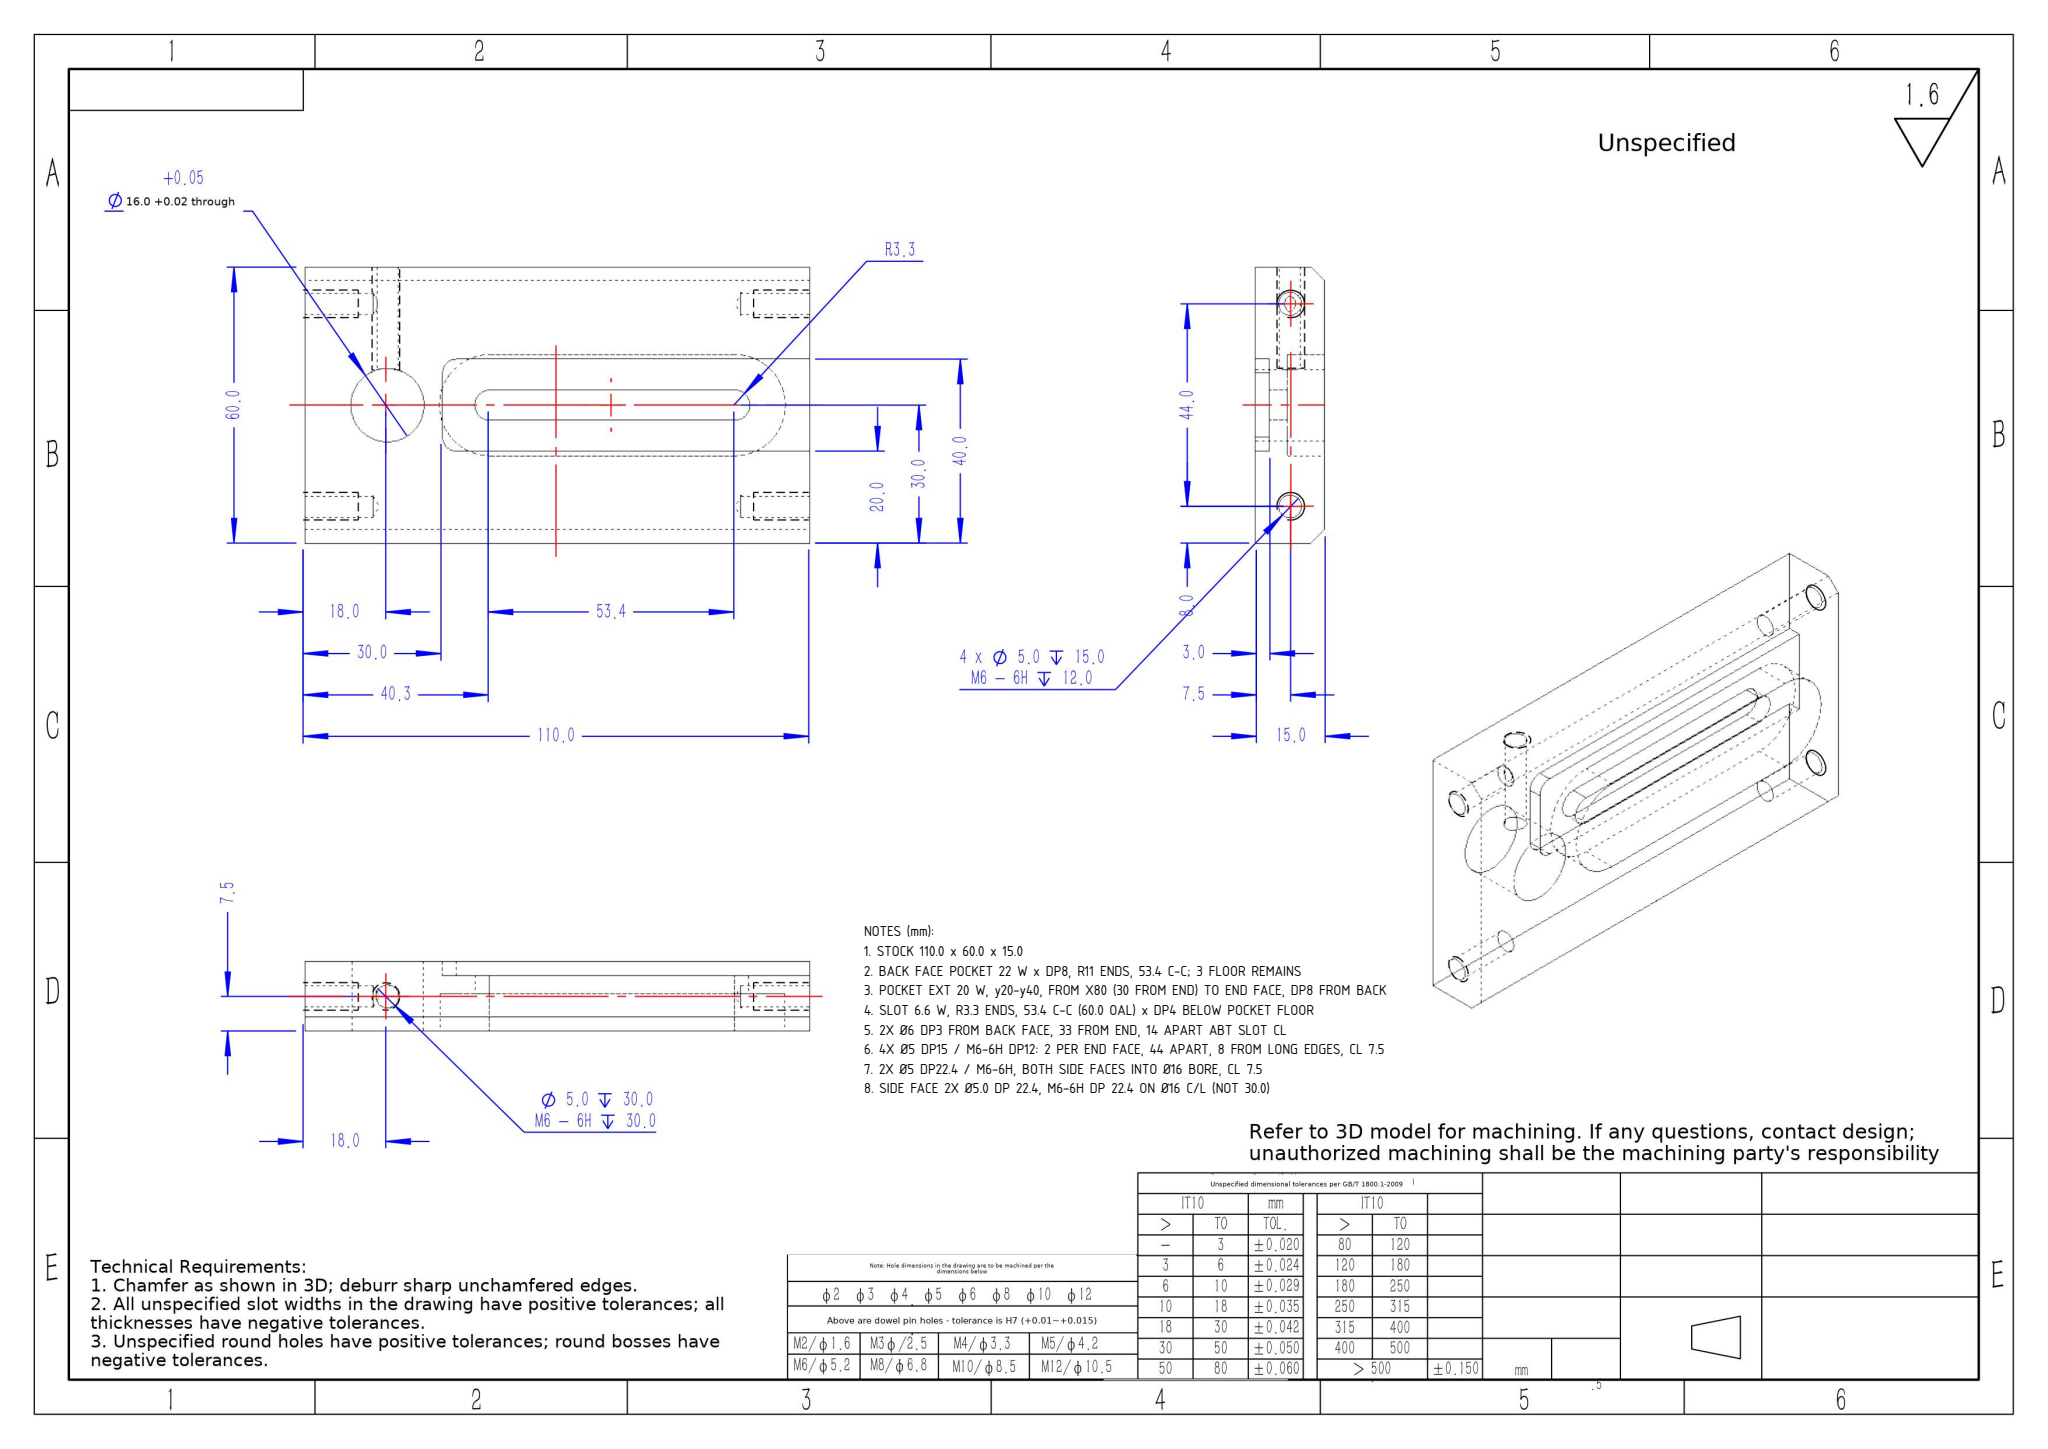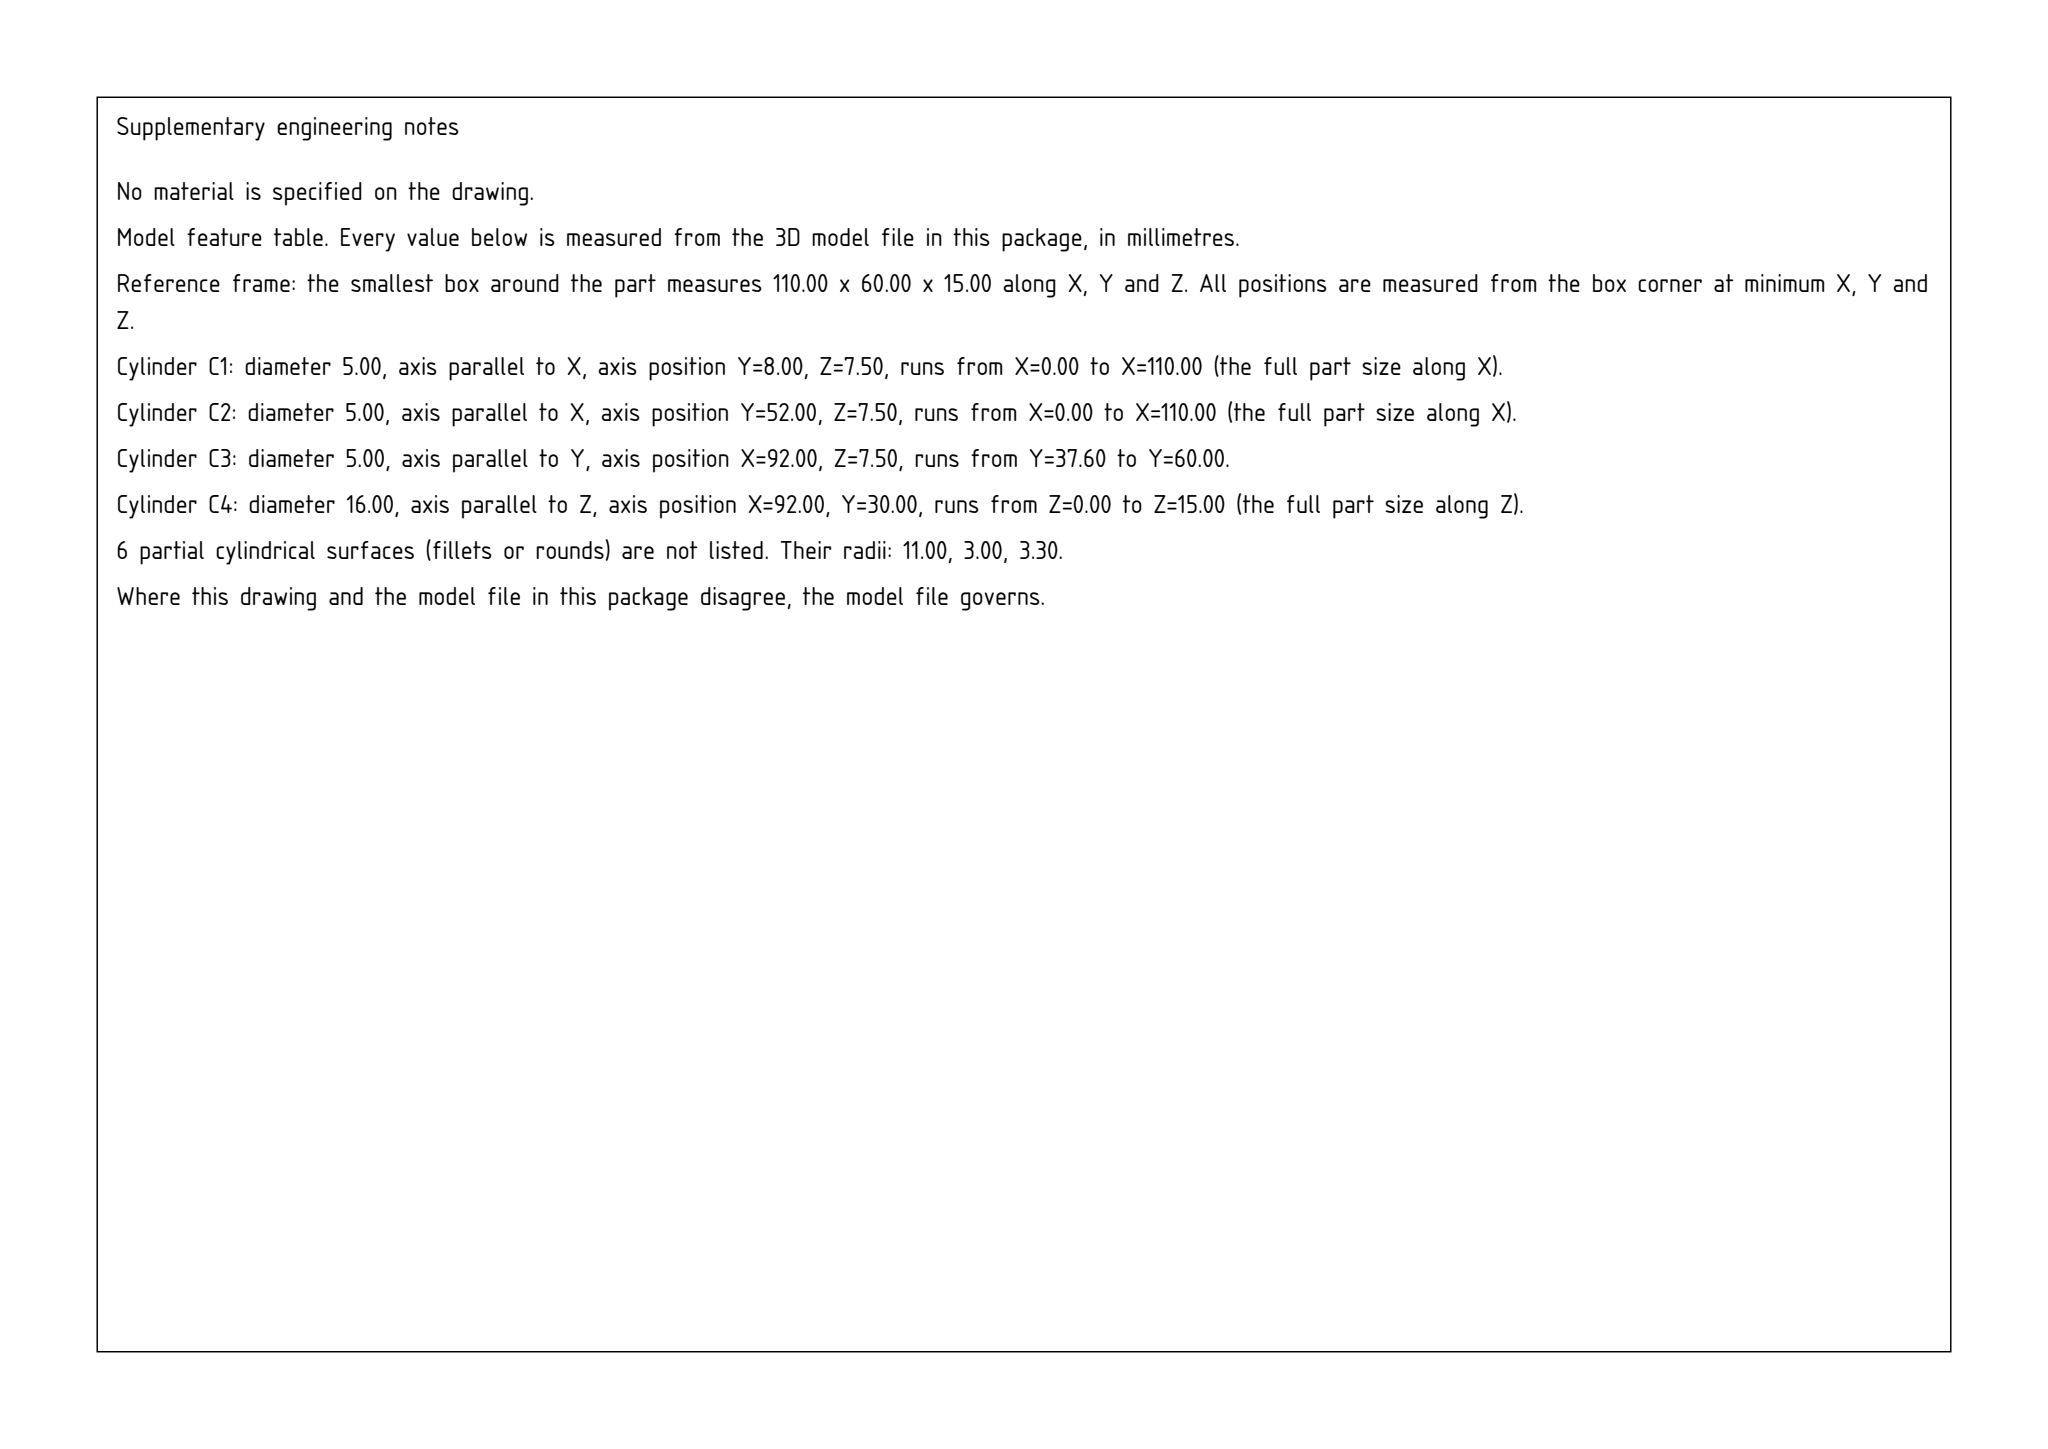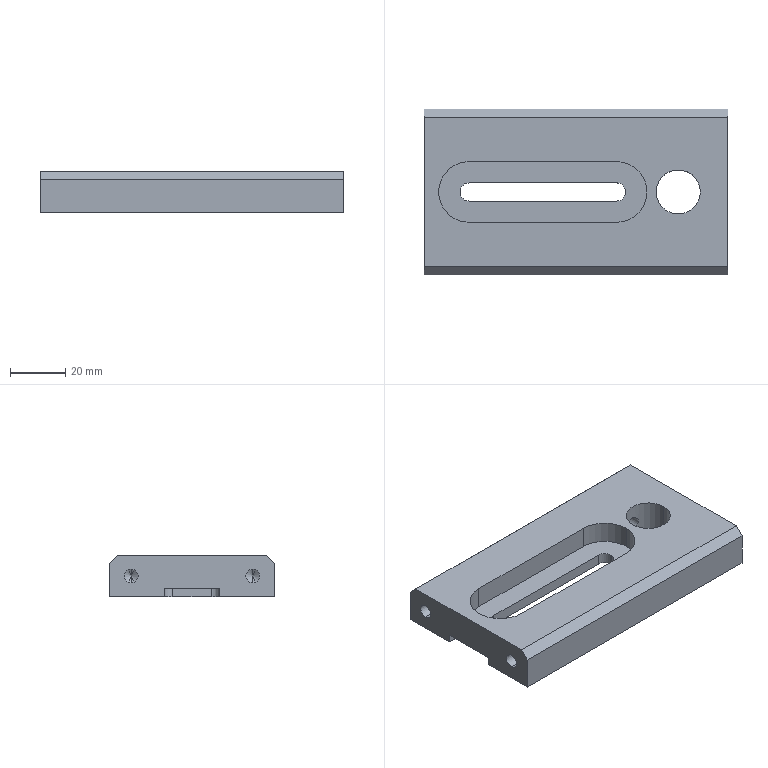Part | SolidWorks | mm | 1 solid | 45 faces | box 110 x 60 x 15 mm | volume 74570 mm3 | cylinder 20 | plane 17 | cone 8 | commonest cylinder face diameters 5 x10 22 x3 6.6 x3 16 x2 6 x2
Drawing notes:
STOCK 110.0 x 60.0 x 15.0 | from the solid: bbox_xyz [110,60,15]
BACK FACE POCKET 22 W x DP8, R11 ENDS, 53.4 C-C; 3 FLOOR REMAINS | from the solid: Ø22 z-cyls x=16.3 & 69.7 dp8; y-planes 19/41; z-planes 15 to 7; floor z0-3
POCKET EXT 20 W, y20-y40, FROM X80 (30 FROM END) TO END FACE, DP8 FROM BACK | from the solid: planes x=80, y=20, y=40; back z=15 to recess floor z=7
SLOT 6.6 W, R3.3 ENDS, 53.4 C-C (60.0 OAL) x DP4 BELOW POCKET FLOOR | from the solid: y-planes 26.7/33.3; Ø6.6 z-cyls x=16.3 & 69.7, z 3-7
2X Ø6 DP3 FROM BACK FACE, 33 FROM END, 14 APART ABT SLOT CL | from the solid: Ø6 z-cyls x=77, y=23 & 37, dp3 (110-77=33; 37-23=14)
4X Ø5 DP15 / M6-6H DP12: 2 PER END FACE, 44 APART, 8 FROM LONG EDGES, CL 7.5 | from the solid: Ø5 x-axis cyls y=8 & 52, z=7.5, len 15, from x=0 and x=110 faces
2X Ø5 DP22.4 / M6-6H, BOTH SIDE FACES INTO Ø16 BORE, CL 7.5 | from the solid: Ø5 y-axis cyls at x=92, z=7.5, len 22.4 from y=0 and y=60
SIDE FACE 2X Ø5.0 DP 22.4, M6-6H DP 22.4 ON Ø16 C/L (NOT 30.0) | from the solid: cylinders dia 5.0 axis x... wait: [5.0,"y",[92.0,null,7.5],22.4,2] - two Ø5 holes along Y at x=92 (Ø16 hole CL), z=7.5, length 22.4